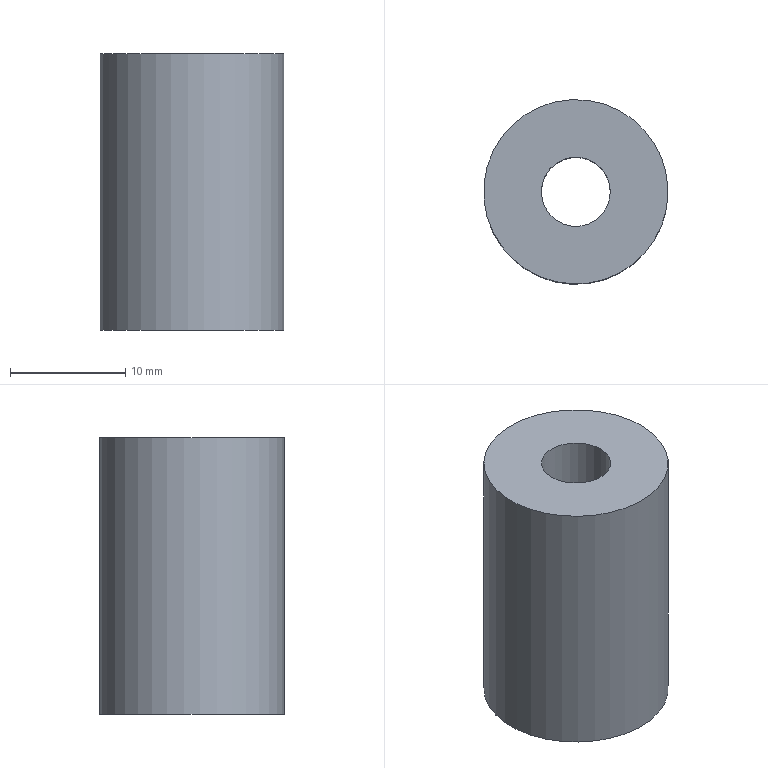Component | NX | COUPLING | 1 solid | 4 faces | box 16 x 16 x 24 mm | volume 4147 mm3 | cylinder 2 | plane 2 | commonest cylinder face diameters 16 x1 6 x1
STEP:
#1=CARTESIAN_POINT('',(0.,0.,0.));
#2=DIRECTION('',(0.,0.,1.));
#3=DIRECTION('',(1.,0.,0.));
#4=AXIS2_PLACEMENT_3D('',#1,#2,#3);
#5=CARTESIAN_POINT('',(633.689,-150.302,-965.));
#6=VERTEX_POINT('',#5);
#7=CARTESIAN_POINT('',(625.689,-150.302,-965.));
#8=DIRECTION('',(0.,0.,1.));
#9=DIRECTION('',(1.,0.,0.));
#10=AXIS2_PLACEMENT_3D('',#7,#8,#9);
#11=CIRCLE('',#10,8.);
#12=CARTESIAN_POINT('',(625.689,-150.302,-965.));
#13=DIRECTION('',(0.,0.,-1.));
#14=DIRECTION('',(-1.,0.,0.));
#15=AXIS2_PLACEMENT_3D('',#12,#13,#14);
#16=CYLINDRICAL_SURFACE('',#15,8.);
#17=CARTESIAN_POINT('',(9.425,0.));
#18=DIRECTION('',(-1.,0.));
#19=VECTOR('',#18,1.);
#20=LINE('',#17,#19);
#21=(GEOMETRIC_REPRESENTATION_CONTEXT(2)PARAMETRIC_REPRESENTATION_CONTEXT()REPRESENTATION_CONTEXT('',''));
#22=DEFINITIONAL_REPRESENTATION('',(#20),#21);
#23=PCURVE('',#16,#22);
#24=CARTESIAN_POINT('',(625.689,-150.302,-965.));
#25=DIRECTION('',(0.,0.,1.));
#26=DIRECTION('',(1.,0.,0.));
#27=AXIS2_PLACEMENT_3D('',#24,#25,#26);
#28=PLANE('',#27);
#29=CARTESIAN_POINT('',(0.,0.));
#30=DIRECTION('',(1.,0.));
#31=AXIS2_PLACEMENT_2D('',#29,#30);
#32=CIRCLE('',#31,8.);
#33=(GEOMETRIC_REPRESENTATION_CONTEXT(2)PARAMETRIC_REPRESENTATION_CONTEXT()REPRESENTATION_CONTEXT('',''));
#34=DEFINITIONAL_REPRESENTATION('',(#32),#33);
#35=PCURVE('',#28,#34);
#36=SURFACE_CURVE('',#11,(#23,#35),.PCURVE_S1.);
#37=EDGE_CURVE('',#6,#6,#36,.T.);
#38=ORIENTED_EDGE('',*,*,#37,.F.);
#39=CARTESIAN_POINT('',(633.689,-150.302,-989.));
#40=VERTEX_POINT('',#39);
#41=CARTESIAN_POINT('',(633.689,-150.302,-965.));
#42=CARTESIAN_POINT('',(633.689,-150.302,-989.));
#43=B_SPLINE_CURVE_WITH_KNOTS('',1,(#41,#42),.UNSPECIFIED.,.F.,.F.,(2,2),(0.,24.),.PIECEWISE_BEZIER_KNOTS.);
#44=CARTESIAN_POINT('',(9.425,0.));
#45=DIRECTION('',(0.,1.));
#46=VECTOR('',#45,1.);
#47=LINE('',#44,#46);
#48=(GEOMETRIC_REPRESENTATION_CONTEXT(2)PARAMETRIC_REPRESENTATION_CONTEXT()REPRESENTATION_CONTEXT('',''));
#49=DEFINITIONAL_REPRESENTATION('',(#47),#48);
#50=PCURVE('',#16,#49);
#51=CARTESIAN_POINT('',(3.142,0.));
#52=DIRECTION('',(0.,1.));
#53=VECTOR('',#52,1.);
#54=LINE('',#51,#53);
#55=(GEOMETRIC_REPRESENTATION_CONTEXT(2)PARAMETRIC_REPRESENTATION_CONTEXT()REPRESENTATION_CONTEXT('',''));
#56=DEFINITIONAL_REPRESENTATION('',(#54),#55);
#57=PCURVE('',#16,#56);
#58=SEAM_CURVE('',#43,(#50,#57),.PCURVE_S1.);
#59=EDGE_CURVE('',#6,#40,#58,.T.);
#60=ORIENTED_EDGE('',*,*,#59,.T.);
#61=CARTESIAN_POINT('',(625.689,-150.302,-989.));
#62=DIRECTION('',(0.,0.,1.));
#63=DIRECTION('',(1.,0.,0.));
#64=AXIS2_PLACEMENT_3D('',#61,#62,#63);
#65=CIRCLE('',#64,8.);
#66=CARTESIAN_POINT('',(9.425,24.));
#67=DIRECTION('',(-1.,0.));
#68=VECTOR('',#67,1.);
#69=LINE('',#66,#68);
#70=(GEOMETRIC_REPRESENTATION_CONTEXT(2)PARAMETRIC_REPRESENTATION_CONTEXT()REPRESENTATION_CONTEXT('',''));
#71=DEFINITIONAL_REPRESENTATION('',(#69),#70);
#72=PCURVE('',#16,#71);
#73=CARTESIAN_POINT('',(625.689,-150.302,-989.));
#74=DIRECTION('',(0.,0.,1.));
#75=DIRECTION('',(1.,0.,0.));
#76=AXIS2_PLACEMENT_3D('',#73,#74,#75);
#77=PLANE('',#76);
#78=CARTESIAN_POINT('',(0.,0.));
#79=DIRECTION('',(1.,0.));
#80=AXIS2_PLACEMENT_2D('',#78,#79);
#81=CIRCLE('',#80,8.);
#82=(GEOMETRIC_REPRESENTATION_CONTEXT(2)PARAMETRIC_REPRESENTATION_CONTEXT()REPRESENTATION_CONTEXT('',''));
#83=DEFINITIONAL_REPRESENTATION('',(#81),#82);
#84=PCURVE('',#77,#83);
#85=SURFACE_CURVE('',#65,(#72,#84),.PCURVE_S1.);
#86=EDGE_CURVE('',#40,#40,#85,.T.);
#87=ORIENTED_EDGE('',*,*,#86,.T.);
#88=ORIENTED_EDGE('',*,*,#59,.F.);
#89=EDGE_LOOP('',(#38,#60,#87,#88));
#90=FACE_BOUND('',#89,.T.);
#91=ADVANCED_FACE('',(#90),#16,.T.);
#92=CARTESIAN_POINT('',(628.689,-150.302,-965.));
#93=VERTEX_POINT('',#92);
#94=CARTESIAN_POINT('',(625.689,-150.302,-965.));
#95=DIRECTION('',(0.,0.,1.));
#96=DIRECTION('',(1.,0.,0.));
#97=AXIS2_PLACEMENT_3D('',#94,#95,#96);
#98=CIRCLE('',#97,3.);
#99=CARTESIAN_POINT('',(625.689,-150.302,-965.));
#100=DIRECTION('',(0.,0.,-1.));
#101=DIRECTION('',(-1.,0.,0.));
#102=AXIS2_PLACEMENT_3D('',#99,#100,#101);
#103=CYLINDRICAL_SURFACE('',#102,3.);
#104=CARTESIAN_POINT('',(9.425,0.));
#105=DIRECTION('',(-1.,0.));
#106=VECTOR('',#105,1.);
#107=LINE('',#104,#106);
#108=(GEOMETRIC_REPRESENTATION_CONTEXT(2)PARAMETRIC_REPRESENTATION_CONTEXT()REPRESENTATION_CONTEXT('',''));
#109=DEFINITIONAL_REPRESENTATION('',(#107),#108);
#110=PCURVE('',#103,#109);
#111=CARTESIAN_POINT('',(0.,0.));
#112=DIRECTION('',(1.,0.));
#113=AXIS2_PLACEMENT_2D('',#111,#112);
#114=CIRCLE('',#113,3.);
#115=(GEOMETRIC_REPRESENTATION_CONTEXT(2)PARAMETRIC_REPRESENTATION_CONTEXT()REPRESENTATION_CONTEXT('',''));
#116=DEFINITIONAL_REPRESENTATION('',(#114),#115);
#117=PCURVE('',#28,#116);
#118=SURFACE_CURVE('',#98,(#110,#117),.PCURVE_S1.);
#119=EDGE_CURVE('',#93,#93,#118,.T.);
#120=ORIENTED_EDGE('',*,*,#119,.F.);
#121=CARTESIAN_POINT('',(628.689,-150.302,-989.));
#122=VERTEX_POINT('',#121);
#123=CARTESIAN_POINT('',(628.689,-150.302,-965.));
#124=CARTESIAN_POINT('',(628.689,-150.302,-989.));
#125=B_SPLINE_CURVE_WITH_KNOTS('',1,(#123,#124),.UNSPECIFIED.,.F.,.F.,(2,2),(0.,24.),.PIECEWISE_BEZIER_KNOTS.);
#126=CARTESIAN_POINT('',(9.425,0.));
#127=DIRECTION('',(0.,1.));
#128=VECTOR('',#127,1.);
#129=LINE('',#126,#128);
#130=(GEOMETRIC_REPRESENTATION_CONTEXT(2)PARAMETRIC_REPRESENTATION_CONTEXT()REPRESENTATION_CONTEXT('',''));
#131=DEFINITIONAL_REPRESENTATION('',(#129),#130);
#132=PCURVE('',#103,#131);
#133=CARTESIAN_POINT('',(3.142,0.));
#134=DIRECTION('',(0.,1.));
#135=VECTOR('',#134,1.);
#136=LINE('',#133,#135);
#137=(GEOMETRIC_REPRESENTATION_CONTEXT(2)PARAMETRIC_REPRESENTATION_CONTEXT()REPRESENTATION_CONTEXT('',''));
#138=DEFINITIONAL_REPRESENTATION('',(#136),#137);
#139=PCURVE('',#103,#138);
#140=SEAM_CURVE('',#125,(#132,#139),.PCURVE_S1.);
#141=EDGE_CURVE('',#93,#122,#140,.T.);
#142=ORIENTED_EDGE('',*,*,#141,.T.);
#143=CARTESIAN_POINT('',(625.689,-150.302,-989.));
#144=DIRECTION('',(0.,0.,1.));
#145=DIRECTION('',(1.,0.,0.));
#146=AXIS2_PLACEMENT_3D('',#143,#144,#145);
#147=CIRCLE('',#146,3.);
#148=CARTESIAN_POINT('',(9.425,24.));
#149=DIRECTION('',(-1.,0.));
#150=VECTOR('',#149,1.);
#151=LINE('',#148,#150);
#152=(GEOMETRIC_REPRESENTATION_CONTEXT(2)PARAMETRIC_REPRESENTATION_CONTEXT()REPRESENTATION_CONTEXT('',''));
#153=DEFINITIONAL_REPRESENTATION('',(#151),#152);
#154=PCURVE('',#103,#153);
#155=CARTESIAN_POINT('',(0.,0.));
#156=DIRECTION('',(1.,0.));
#157=AXIS2_PLACEMENT_2D('',#155,#156);
#158=CIRCLE('',#157,3.);
#159=(GEOMETRIC_REPRESENTATION_CONTEXT(2)PARAMETRIC_REPRESENTATION_CONTEXT()REPRESENTATION_CONTEXT('',''));
#160=DEFINITIONAL_REPRESENTATION('',(#158),#159);
#161=PCURVE('',#77,#160);
#162=SURFACE_CURVE('',#147,(#154,#161),.PCURVE_S1.);
#163=EDGE_CURVE('',#122,#122,#162,.T.);
#164=ORIENTED_EDGE('',*,*,#163,.T.);
#165=ORIENTED_EDGE('',*,*,#141,.F.);
#166=EDGE_LOOP('',(#120,#142,#164,#165));
#167=FACE_BOUND('',#166,.F.);
#168=ADVANCED_FACE('',(#167),#103,.F.);
#169=ORIENTED_EDGE('',*,*,#37,.T.);
#170=EDGE_LOOP('',(#169));
#171=FACE_BOUND('',#170,.T.);
#172=ORIENTED_EDGE('',*,*,#119,.F.);
#173=EDGE_LOOP('',(#172));
#174=FACE_BOUND('',#173,.T.);
#175=ADVANCED_FACE('',(#171,#174),#28,.T.);
#176=ORIENTED_EDGE('',*,*,#86,.F.);
#177=EDGE_LOOP('',(#176));
#178=FACE_BOUND('',#177,.T.);
#179=ORIENTED_EDGE('',*,*,#163,.T.);
#180=EDGE_LOOP('',(#179));
#181=FACE_BOUND('',#180,.T.);
#182=ADVANCED_FACE('',(#178,#181),#77,.F.);
#183=CLOSED_SHELL('',(#91,#168,#175,#182));
#184=MANIFOLD_SOLID_BREP('',#183);
#185=(LENGTH_UNIT()NAMED_UNIT(*)SI_UNIT(.MILLI.,.METRE.));
#186=UNCERTAINTY_MEASURE_WITH_UNIT(LENGTH_MEASURE(0.00001),#185,'','');
#187=(NAMED_UNIT(*)PLANE_ANGLE_UNIT()SI_UNIT($,.RADIAN.));
#188=(NAMED_UNIT(*)SI_UNIT($,.STERADIAN.)SOLID_ANGLE_UNIT());
#189=(GEOMETRIC_REPRESENTATION_CONTEXT(3)GLOBAL_UNCERTAINTY_ASSIGNED_CONTEXT((#186))GLOBAL_UNIT_ASSIGNED_CONTEXT((#185,#187,#188))REPRESENTATION_CONTEXT('',''));
#190=ADVANCED_BREP_SHAPE_REPRESENTATION('',(#4,#184),#189);